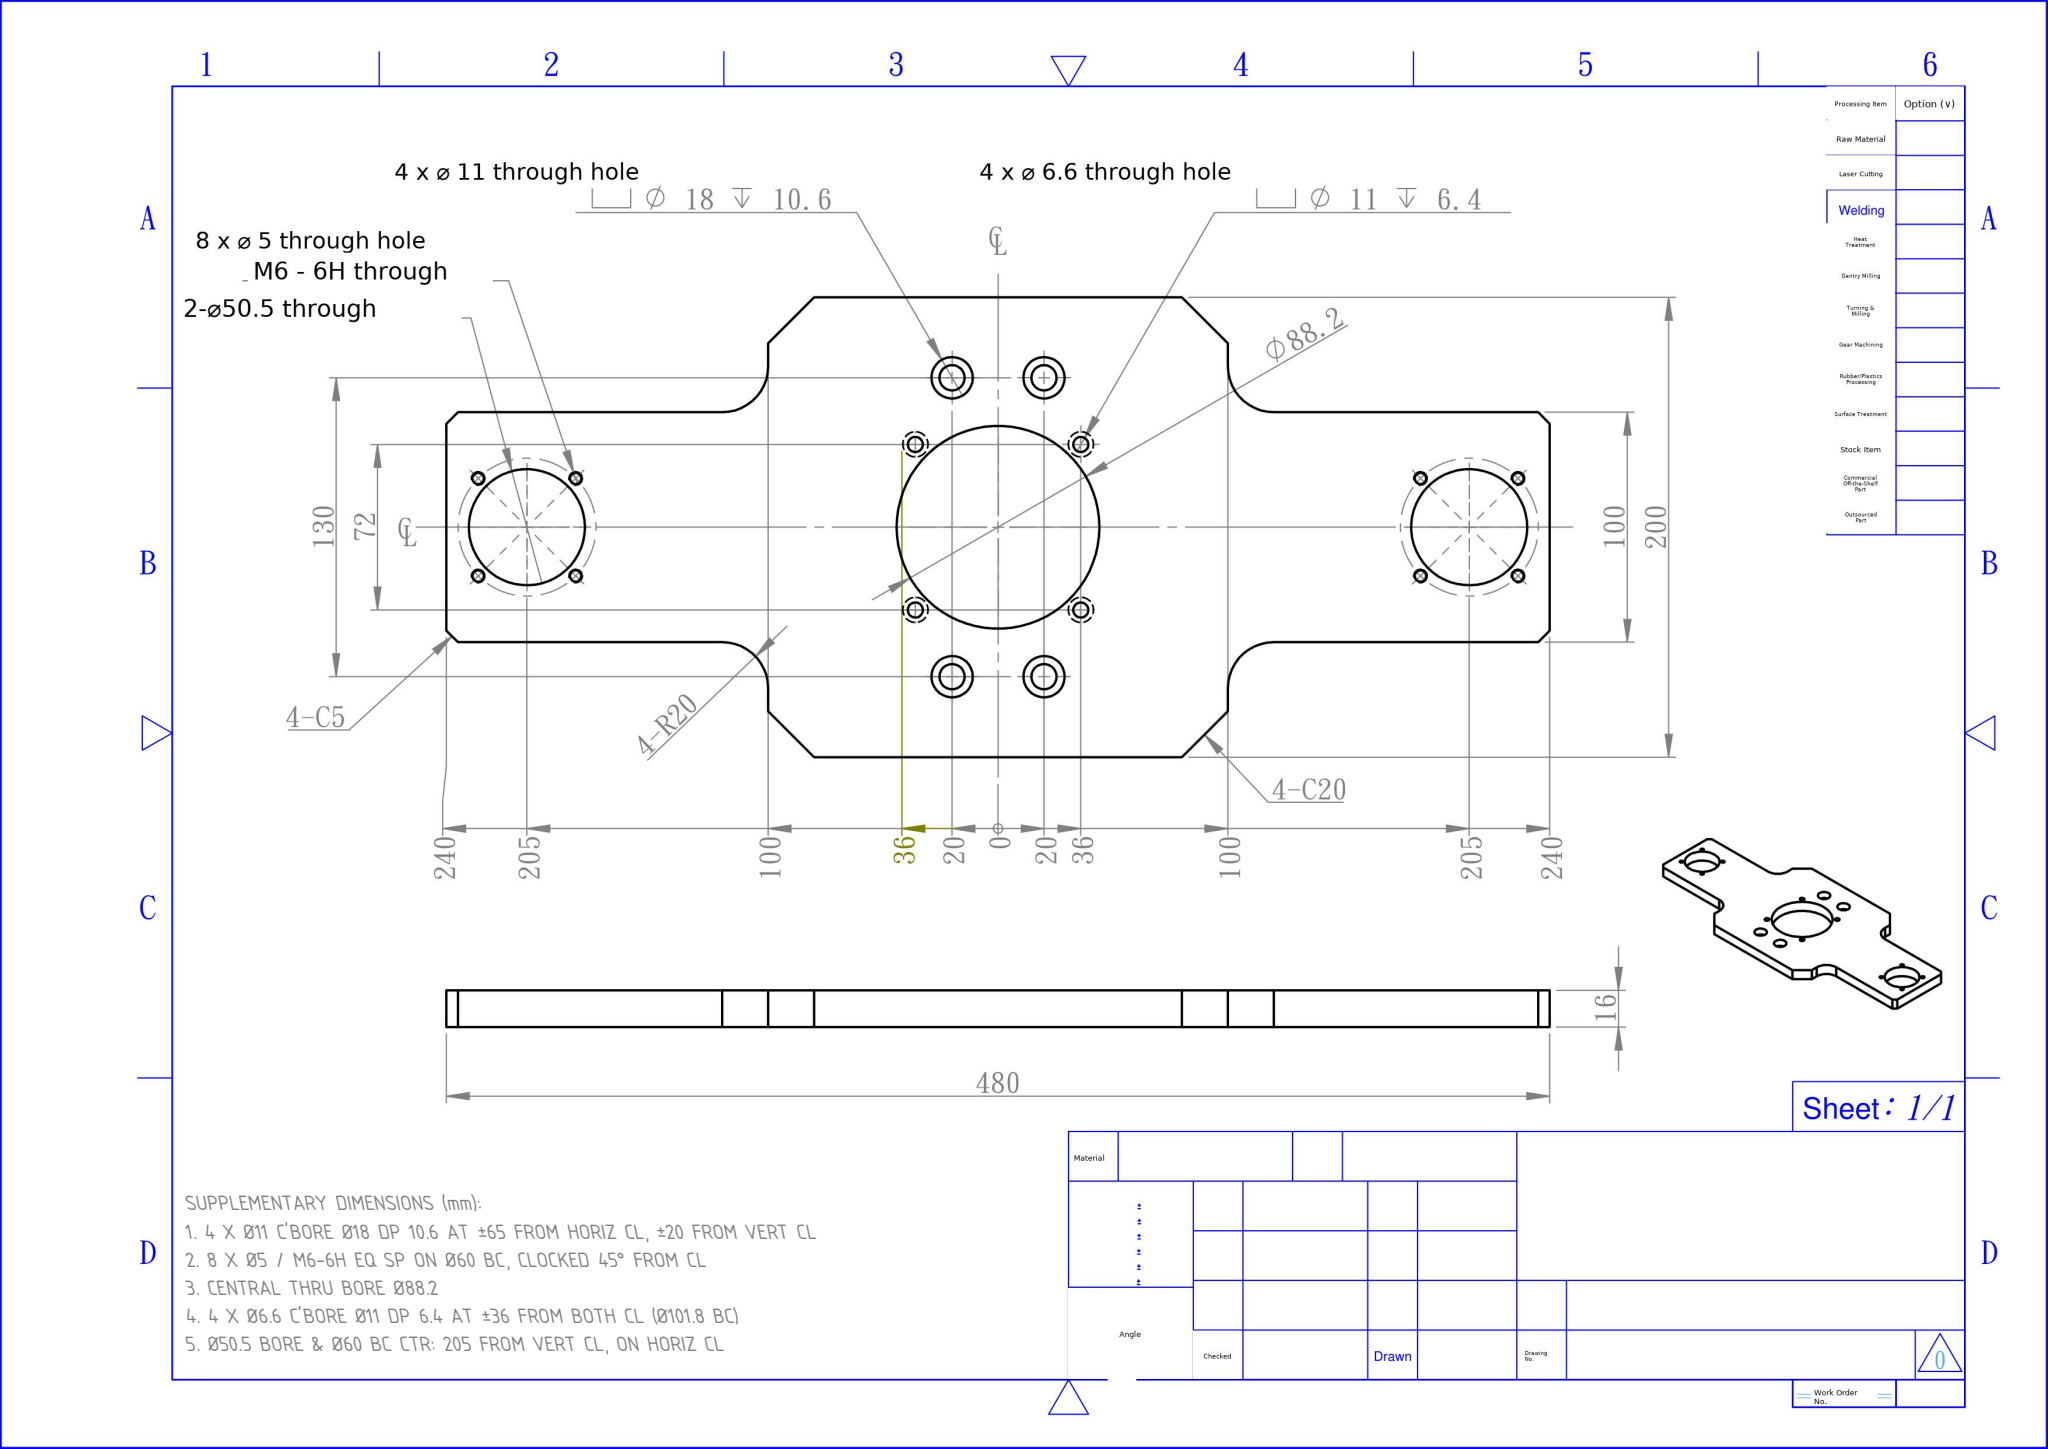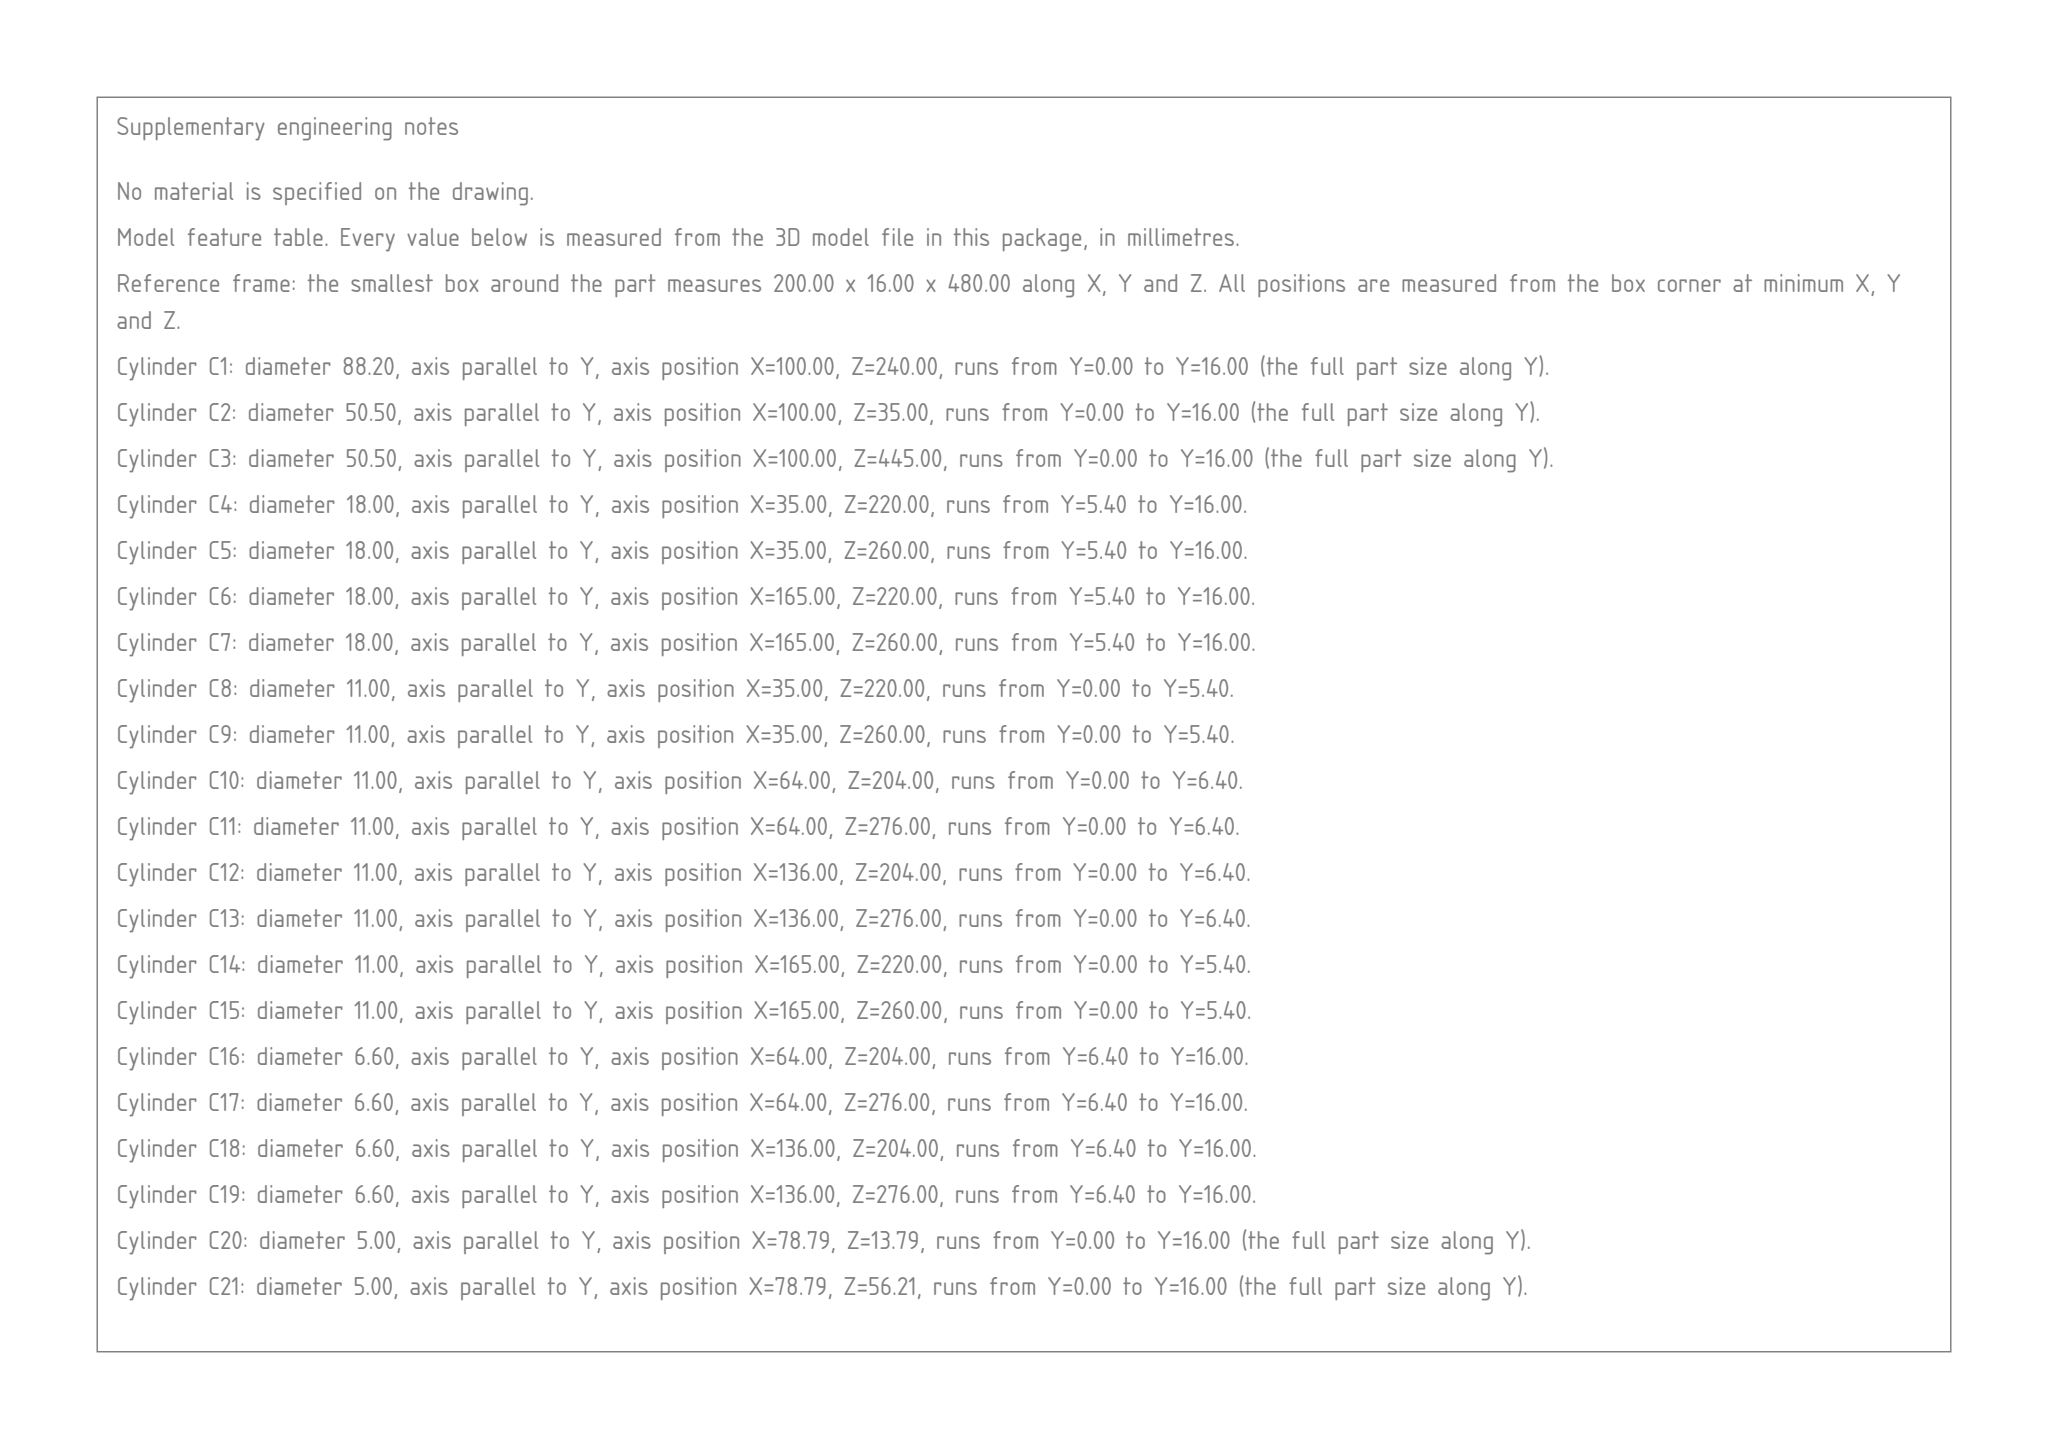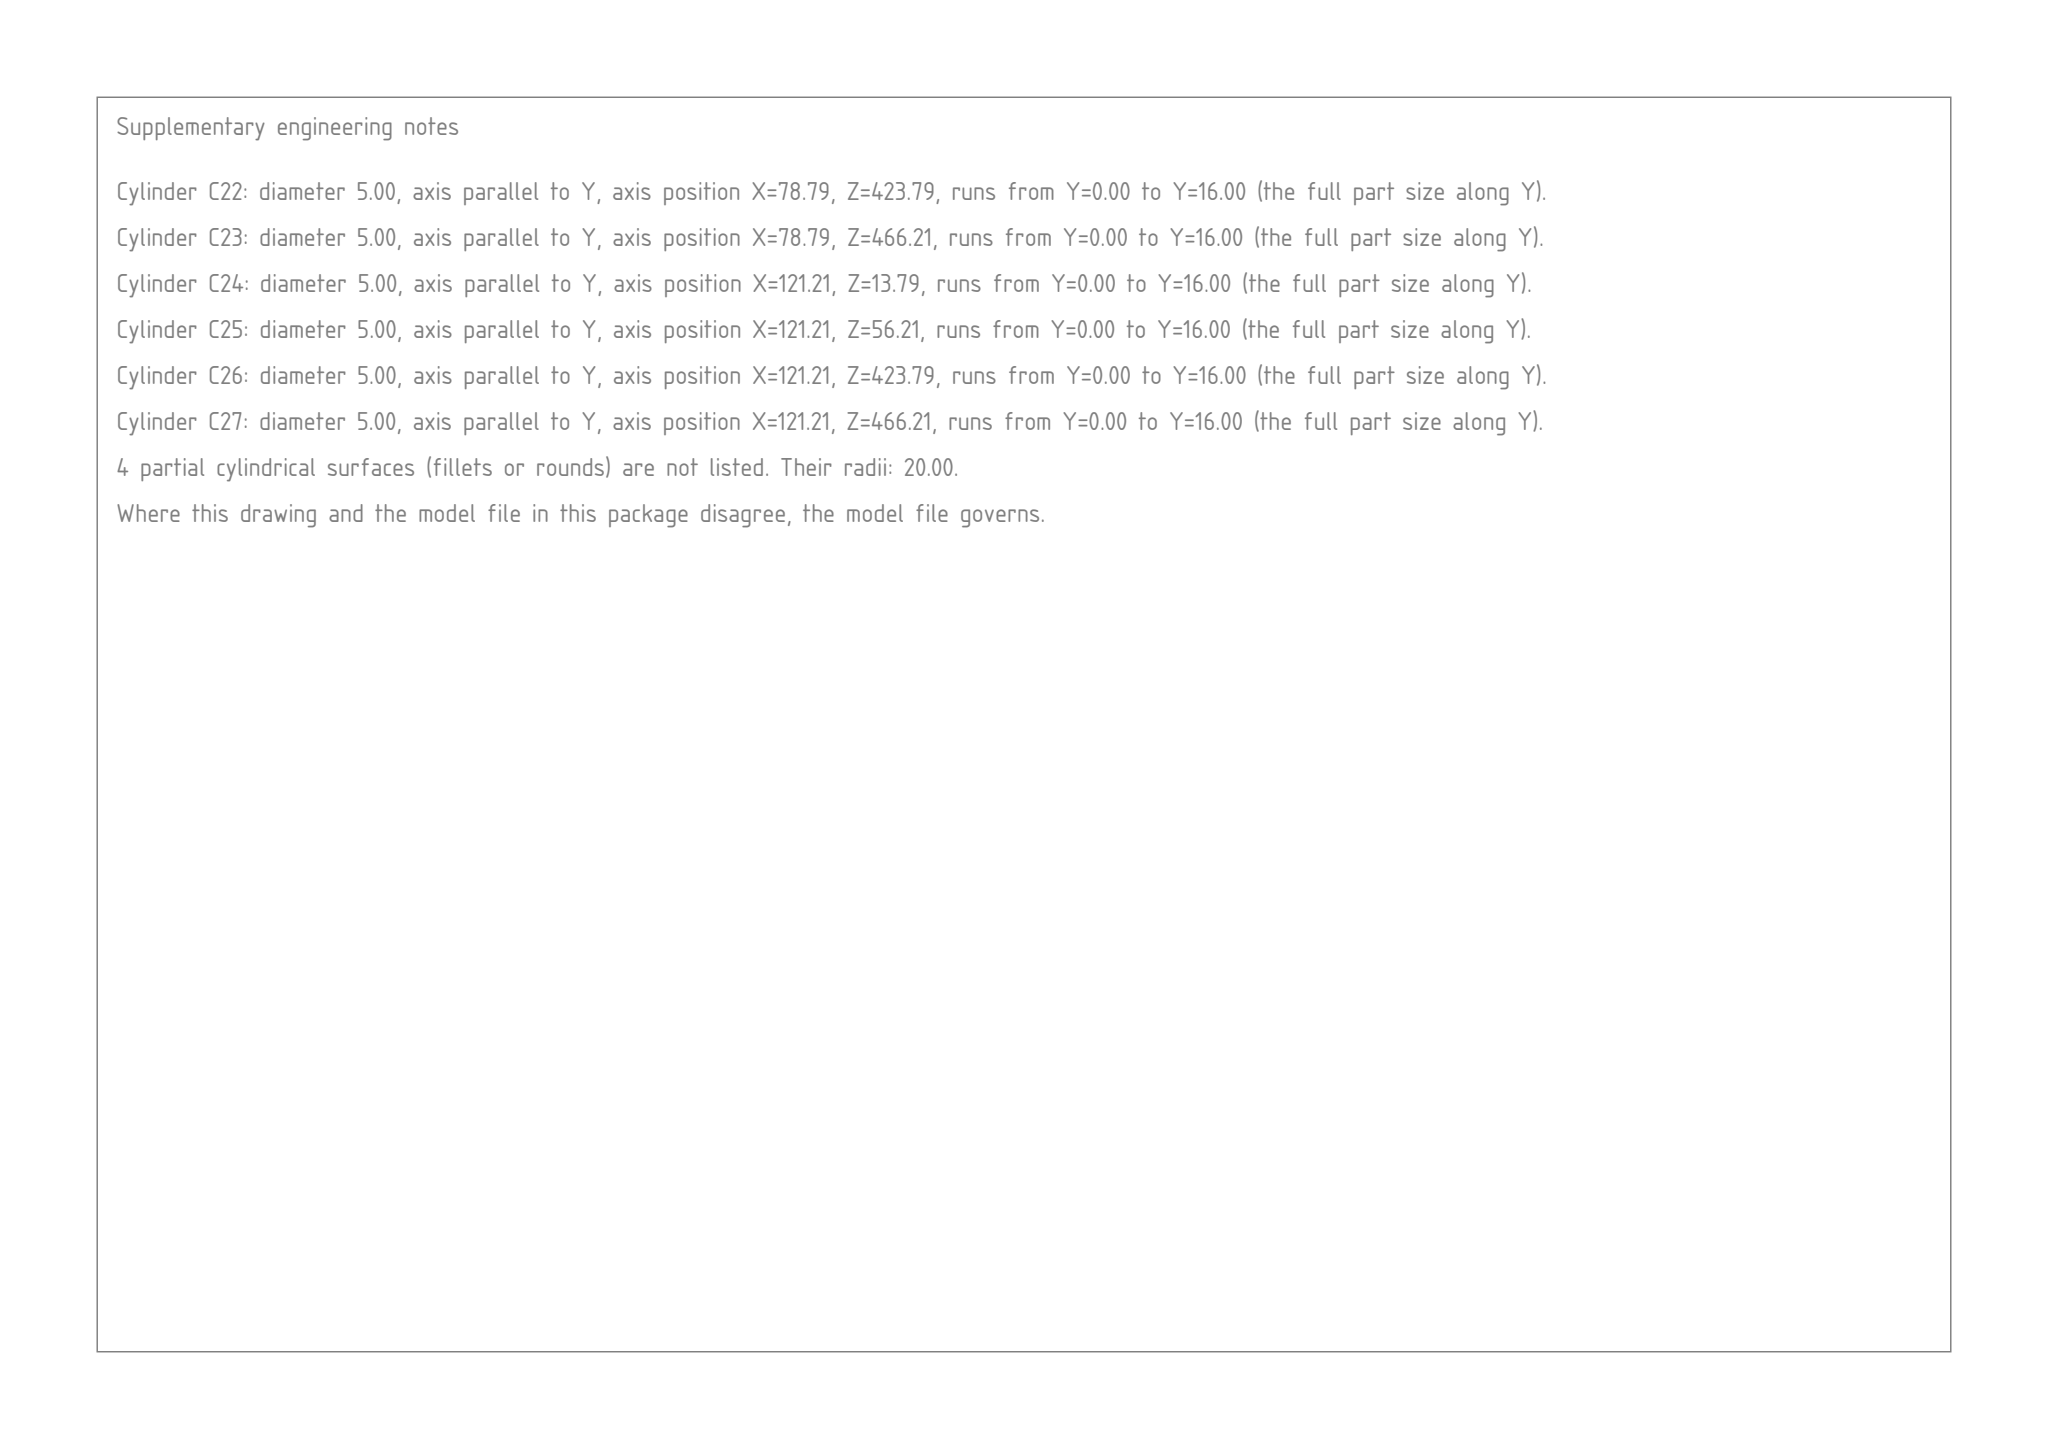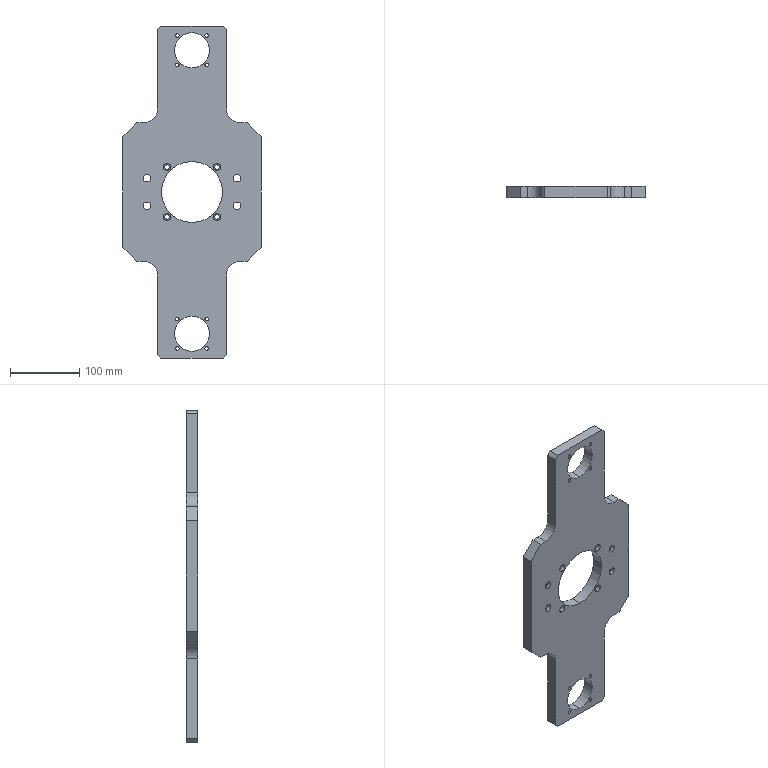Part | SolidWorks | mm | 1 solid | 88 faces | box 200 x 16 x 480 mm | volume 898940 mm3 | cylinder 58 | plane 30 | commonest cylinder face diameters 5 x16 11 x16 18 x8 6.6 x8 50.5 x4 40 x4 88.2 x2
build123d program:
from build123d import *

# Parameters (mm, degrees)
SKETCH1_W                                            = 200
SKETCH1_H                                            = 480
BOSS_EXTRUDE1_DEPTH                                  = 16
SKETCH7_W                                            = 50
SKETCH7_H                                            = 140
CUT_EXTRUDE2_DEPTH                                   = 261.492
CHAMFER1_SIZE                                        = 20
FILLET1_R                                            = 20
SKETCH6_R                                            = 44.1
CUT_EXTRUDE1_DEPTH                                   = 261.492
COUNTERBORE_FOR_M6_HEX_SOCKET_HEAD_CAP_S_D           = 6.6
COUNTERBORE_FOR_M6_HEX_SOCKET_HEAD_CAP_S_CBORE_D     = 11
COUNTERBORE_FOR_M6_HEX_SOCKET_HEAD_CAP_S_CBORE_DEPTH = 6.4
COUNTERBORE_FOR_M10_HEX_SOCKET_HEAD_CAP_D            = 11
COUNTERBORE_FOR_M10_HEX_SOCKET_HEAD_CAP_CBORE_D      = 18
COUNTERBORE_FOR_M10_HEX_SOCKET_HEAD_CAP_CBORE_DEPTH  = 10.6
SKETCH8_R                                            = 25.25
CUT_EXTRUDE3_DEPTH                                   = 261.492
CHAMFER2_SIZE                                        = 5
M6_THREADED_HOLE1_D                                  = 5


with BuildPart() as part:
    # Sketch1 → Boss-Extrude1 (new body)
    with BuildSketch(Plane(origin=(0, 0, 0), x_dir=(1, 0, 0), z_dir=(0, 1, 0))):
        Rectangle(SKETCH1_W, SKETCH1_H)
    extrude(amount=BOSS_EXTRUDE1_DEPTH)

    # Sketch7 → Cut-Extrude2 (cut, through all)
    with BuildSketch(Plane(origin=(0, 16, 0), x_dir=(1, 0, 0), z_dir=(0, 1, 0))):
        with Locations((75, 170)):
            Rectangle(SKETCH7_W, SKETCH7_H)
        with Locations((-75, 170)):
            Rectangle(SKETCH7_W, SKETCH7_H)
        with Locations((75, -170)):
            Rectangle(SKETCH7_W, SKETCH7_H)
        with Locations((-75, -170)):
            Rectangle(SKETCH7_W, SKETCH7_H)
    extrude(amount=-CUT_EXTRUDE2_DEPTH, mode=Mode.SUBTRACT)

    # Chamfer1
    chamfer1_edges = [part.edges().sort_by_distance(p)[0] for p in [
        (-100, 8, -100),
        (100, 8, 100),
        (-100, 8, 100),
        (100, 8, -100),
    ]]
    chamfer(chamfer1_edges, length=CHAMFER1_SIZE)

    # Fillet1
    fillet1_edges = [part.edges().sort_by_distance(p)[0] for p in [
        (-50, 8, -100),
        (50, 8, 100),
        (-50, 8, 100),
        (50, 8, -100),
    ]]
    fillet(fillet1_edges, radius=FILLET1_R)

    # Sketch6 → Cut-Extrude1 (cut, through all)
    with BuildSketch(Plane(origin=(0, 16, 0), x_dir=(1, 0, 0), z_dir=(0, 1, 0))):
        with Locations(Location((0, 0, 0), (0, 0, 270))):
            Circle(SKETCH6_R)
    extrude(amount=-CUT_EXTRUDE1_DEPTH, mode=Mode.SUBTRACT)

    # Counterbore for M6 Hex Socket Head Cap S (through all)
    with Locations(Plane.XZ):
        with Locations((-36, -36), (-36, 36), (36, 36), (36, -36)):
            CounterBoreHole(COUNTERBORE_FOR_M6_HEX_SOCKET_HEAD_CAP_S_D / 2, COUNTERBORE_FOR_M6_HEX_SOCKET_HEAD_CAP_S_CBORE_D / 2, COUNTERBORE_FOR_M6_HEX_SOCKET_HEAD_CAP_S_CBORE_DEPTH)

    # Counterbore for M10 Hex Socket Head Cap (through all)
    with Locations(Plane(origin=(0, 16, 0), x_dir=(1, 0, 0), z_dir=(0, 1, 0))):
        with Locations((-65, 20), (-65, -20), (65, -20), (65, 20)):
            CounterBoreHole(COUNTERBORE_FOR_M10_HEX_SOCKET_HEAD_CAP_D / 2, COUNTERBORE_FOR_M10_HEX_SOCKET_HEAD_CAP_CBORE_D / 2, COUNTERBORE_FOR_M10_HEX_SOCKET_HEAD_CAP_CBORE_DEPTH)

    # Sketch8 → Cut-Extrude3 (cut, through all)
    with BuildSketch(Plane(origin=(0, 16, 0), x_dir=(1, 0, 0), z_dir=(0, 1, 0))):
        with Locations(Location((0, 205, 0), (0, 0, 270))):
            Circle(SKETCH8_R)
        with Locations(Location((0, -205, 0), (0, 0, 270))):
            Circle(SKETCH8_R)
    extrude(amount=-CUT_EXTRUDE3_DEPTH, mode=Mode.SUBTRACT)

    # Chamfer2
    chamfer2_edges = [part.edges().sort_by_distance(p)[0] for p in [
        (-50, 8, -240),
        (50, 8, 240),
        (-50, 8, 240),
        (50, 8, -240),
    ]]
    chamfer(chamfer2_edges, length=CHAMFER2_SIZE)

    # M6 Threaded Hole1 (through all)
    with Locations(Plane(origin=(0, 16, 0), x_dir=(1, 0, 0), z_dir=(0, 1, 0))):
        with Locations((-21.213, -226.213), (21.213, -226.213), (21.213, -183.787), (-21.213, -183.787), (-21.213, 183.787), (21.213, 183.787), (21.213, 226.213), (-21.213, 226.213)):
            Hole(M6_THREADED_HOLE1_D / 2)


solid = part.part